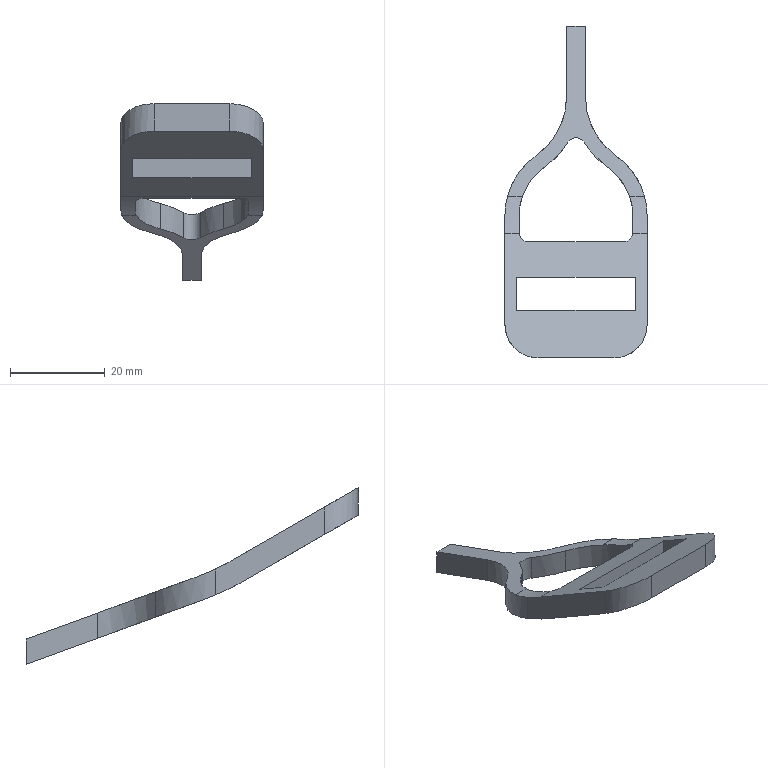Component | NX | BLADE | 1 solid | 33 faces | volume 4533 mm3 | plane 17 | cylinder 16 | commonest cylinder face diameters 4 x3 100 x2 14 x2 31.077 x2 30 x2 36 x2 25.077 x2 110 x1